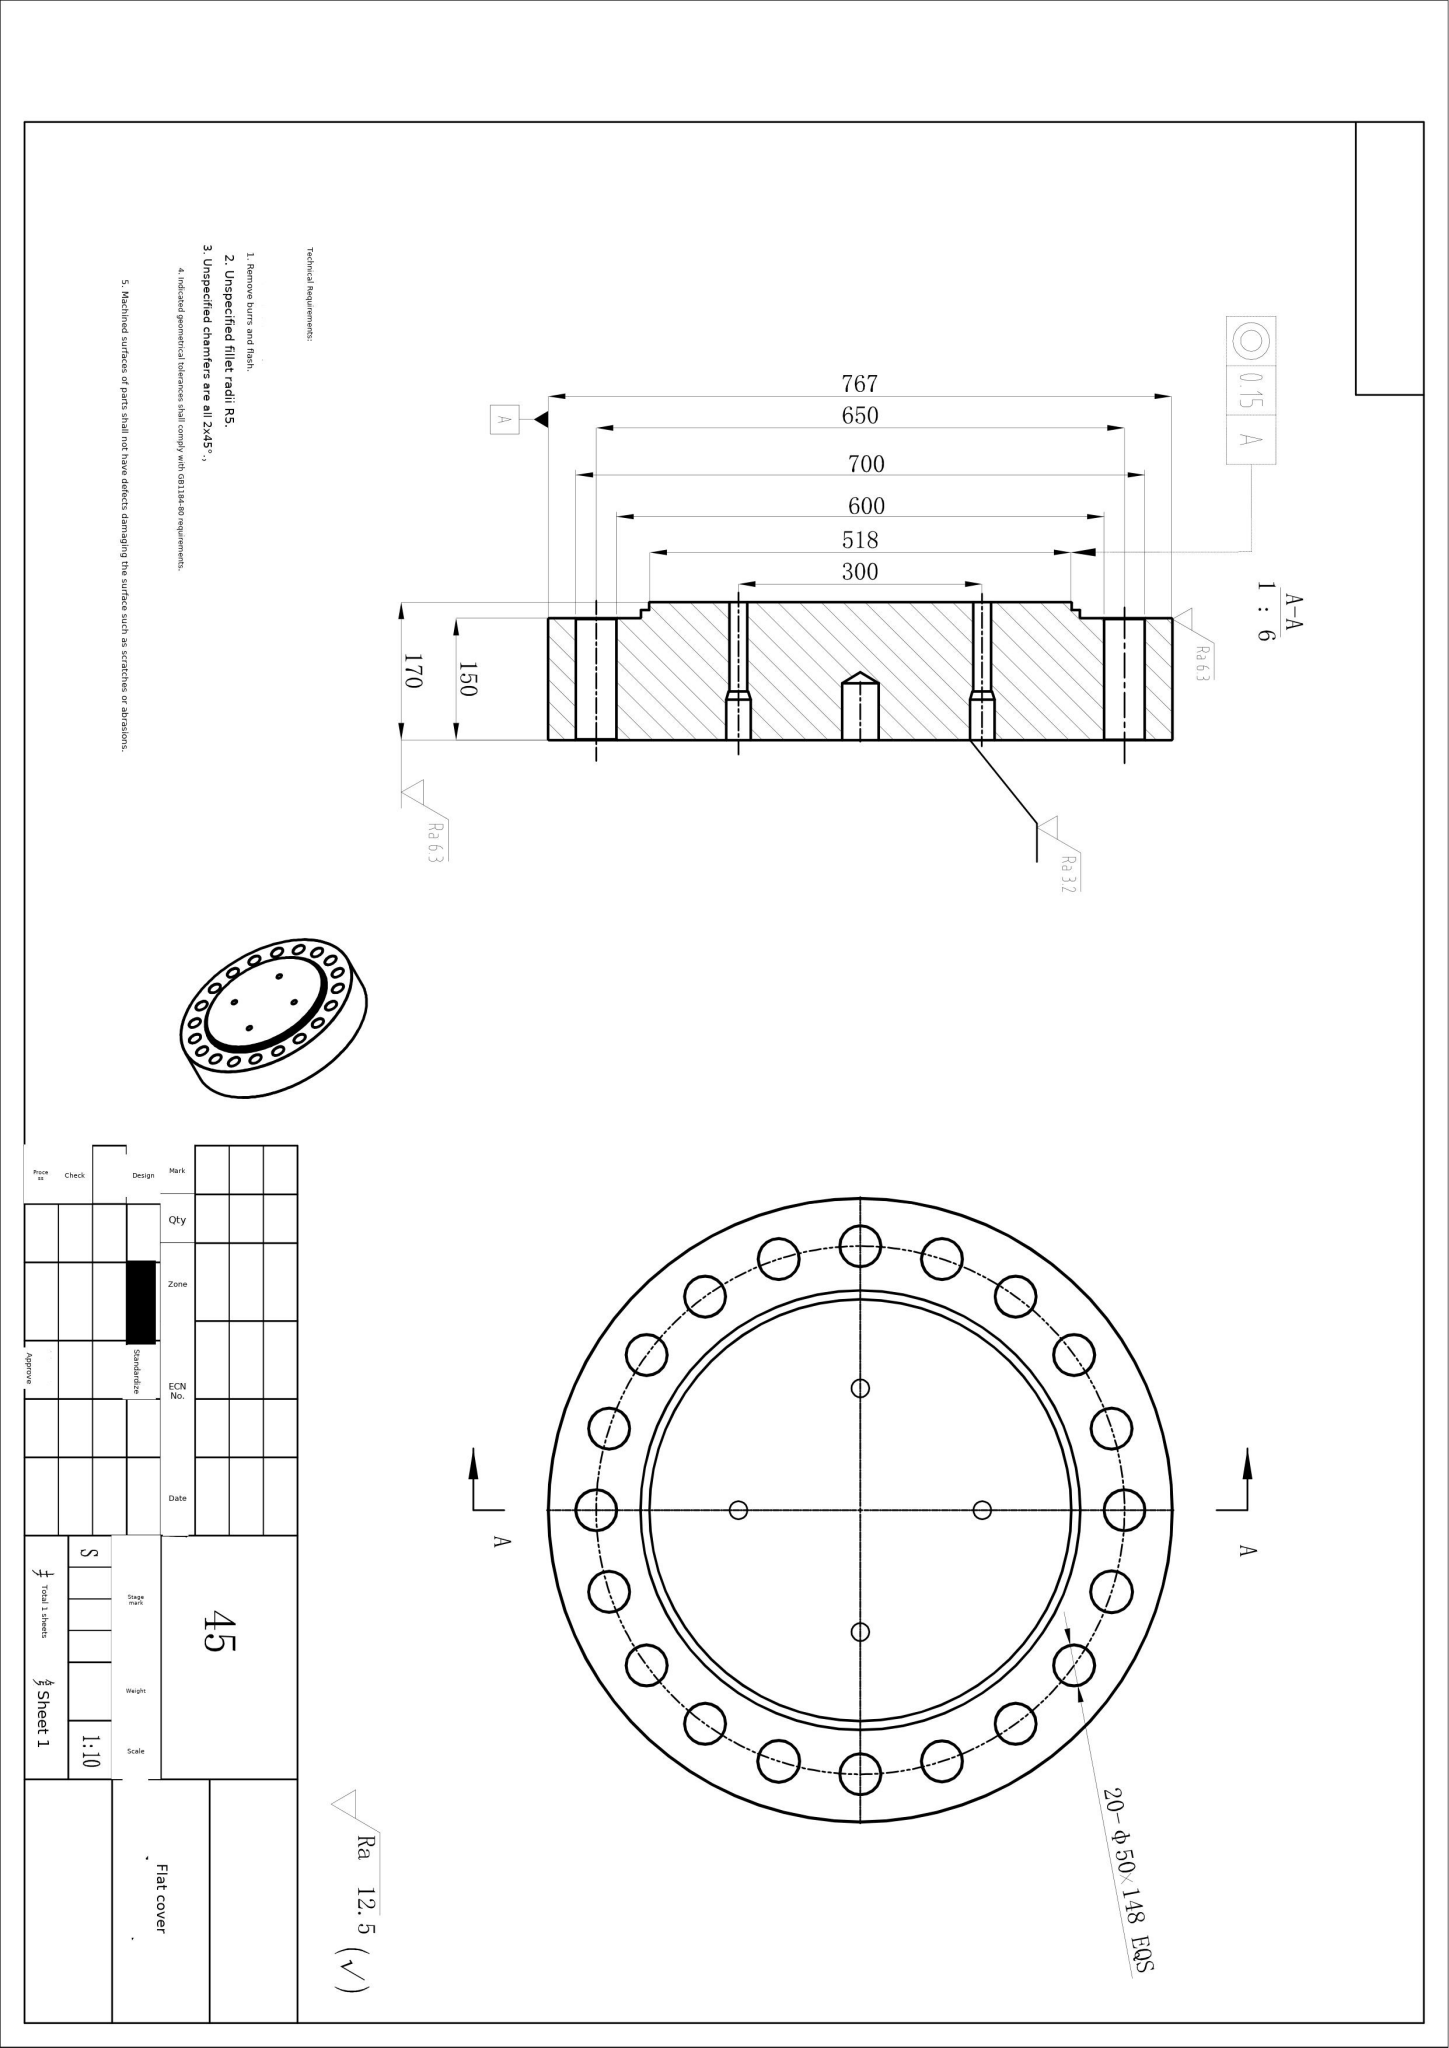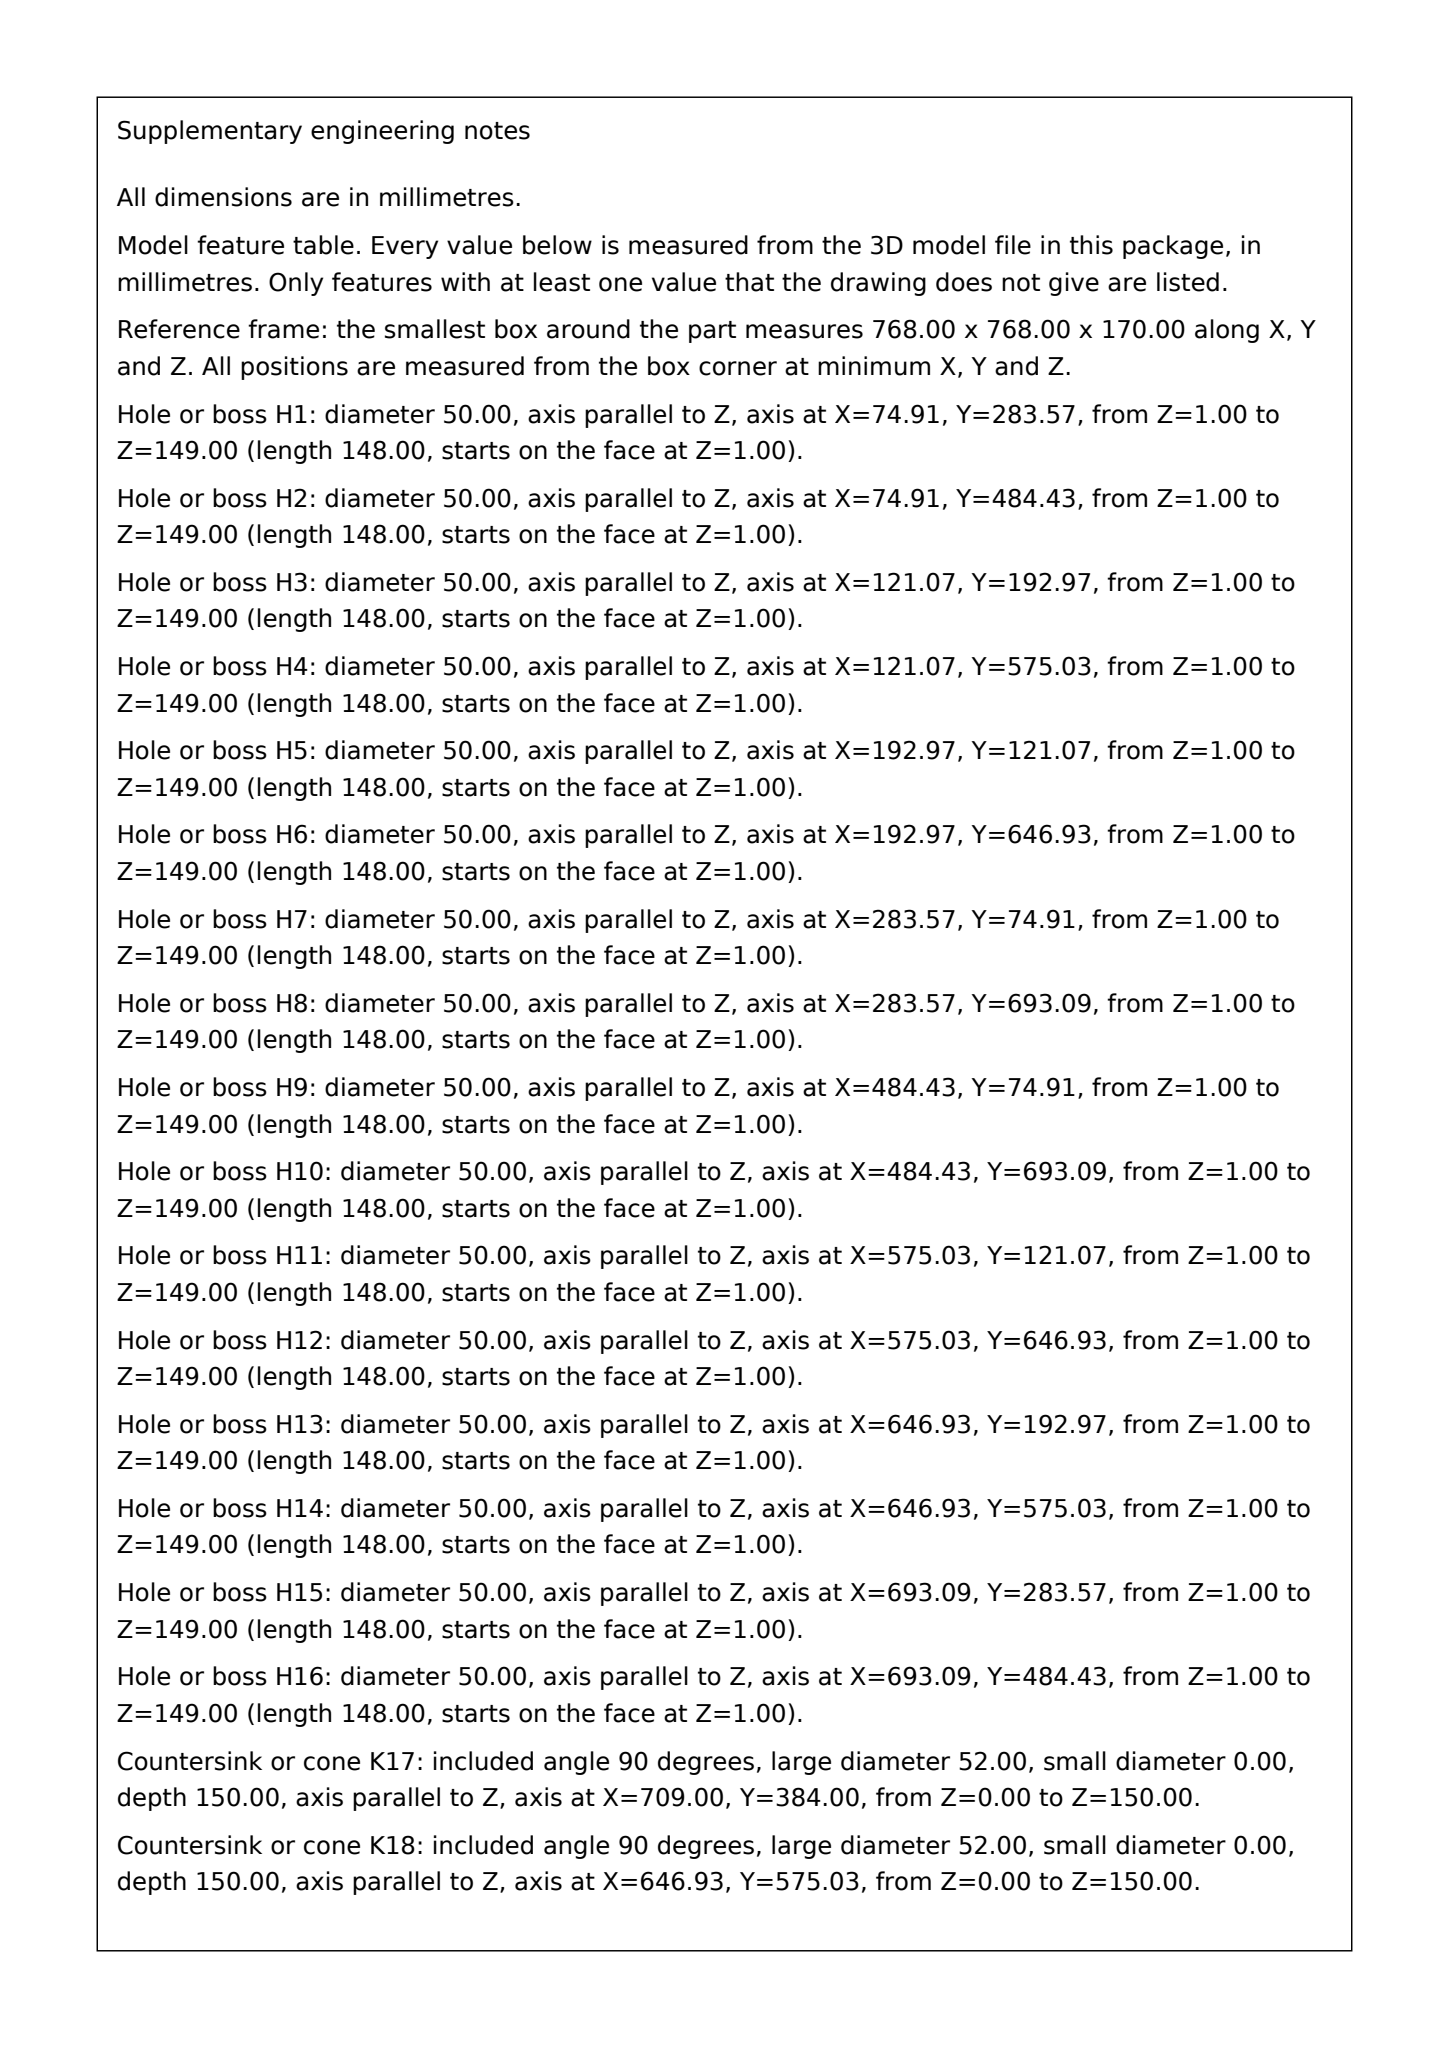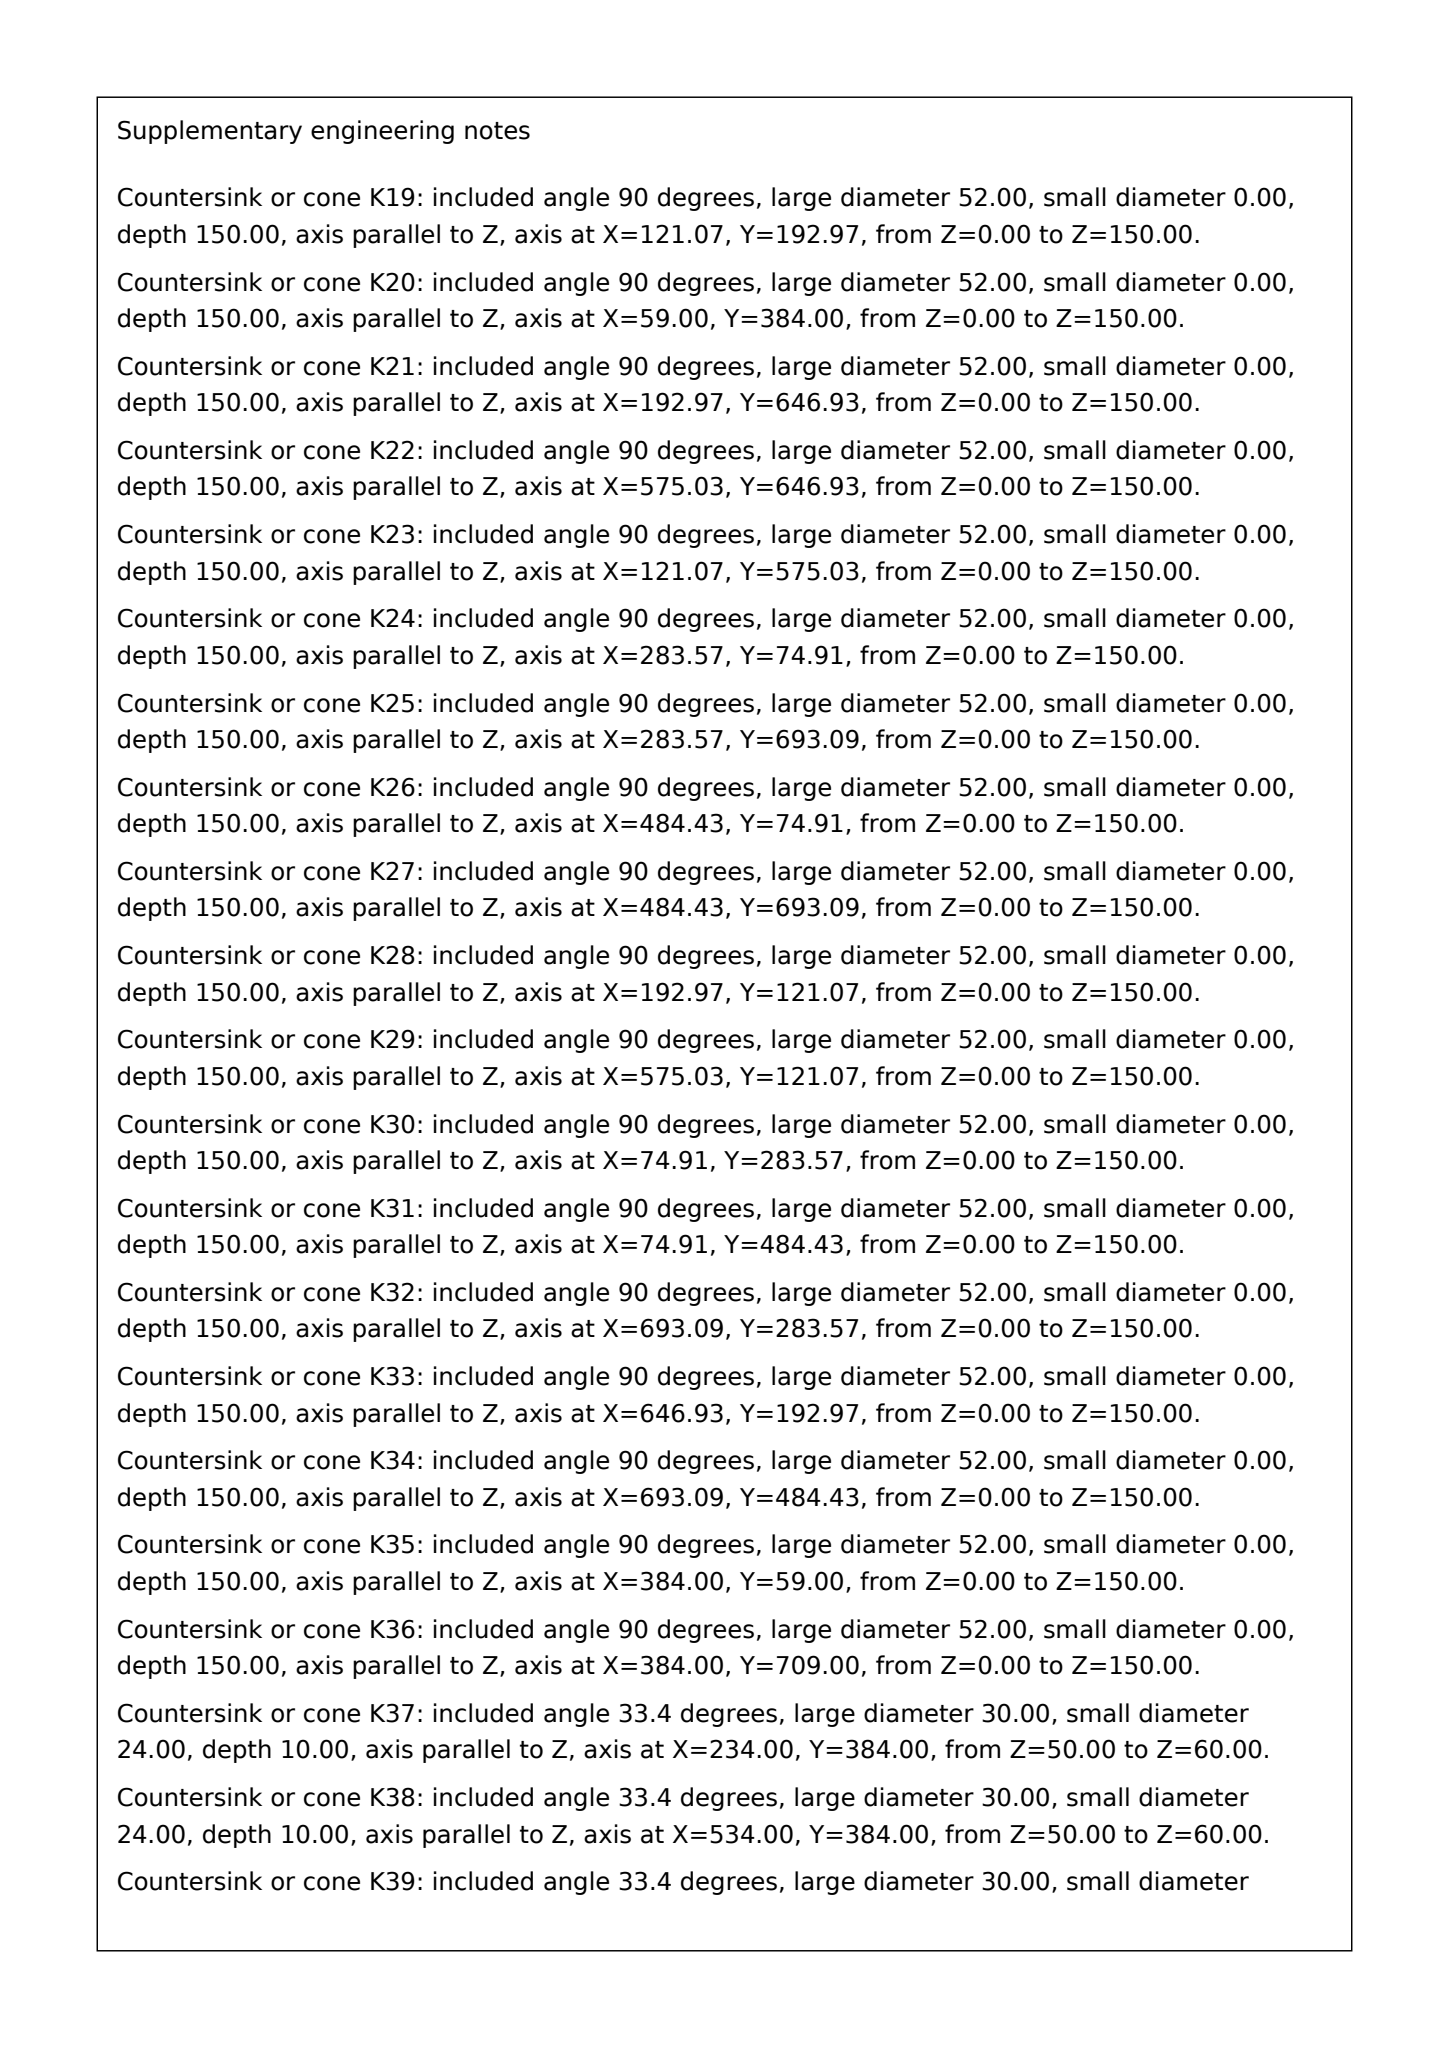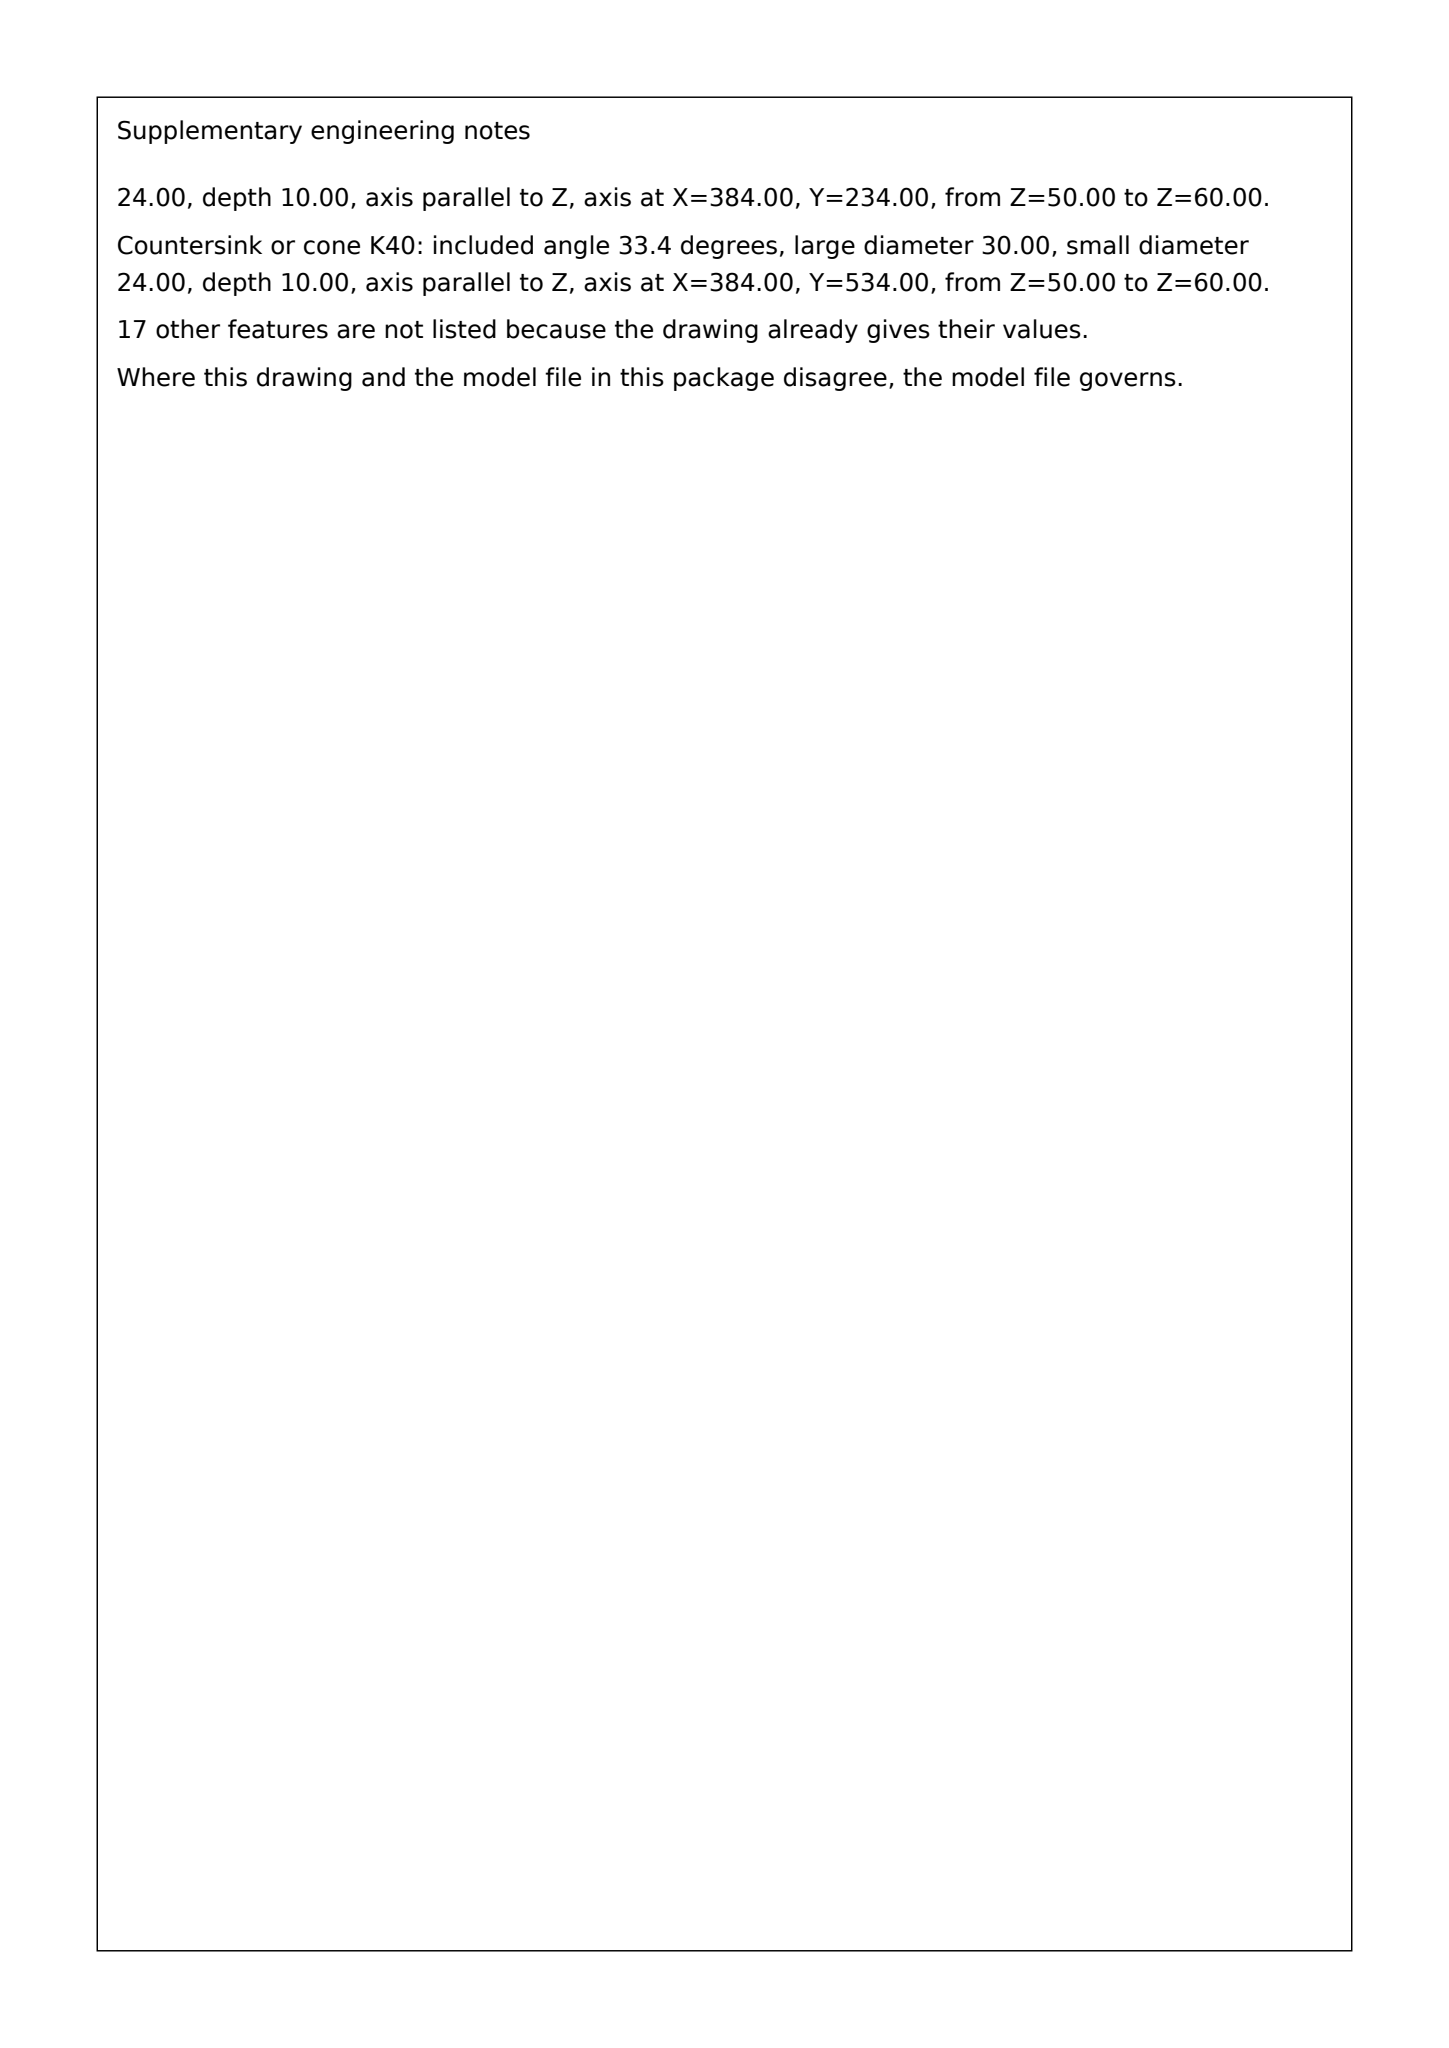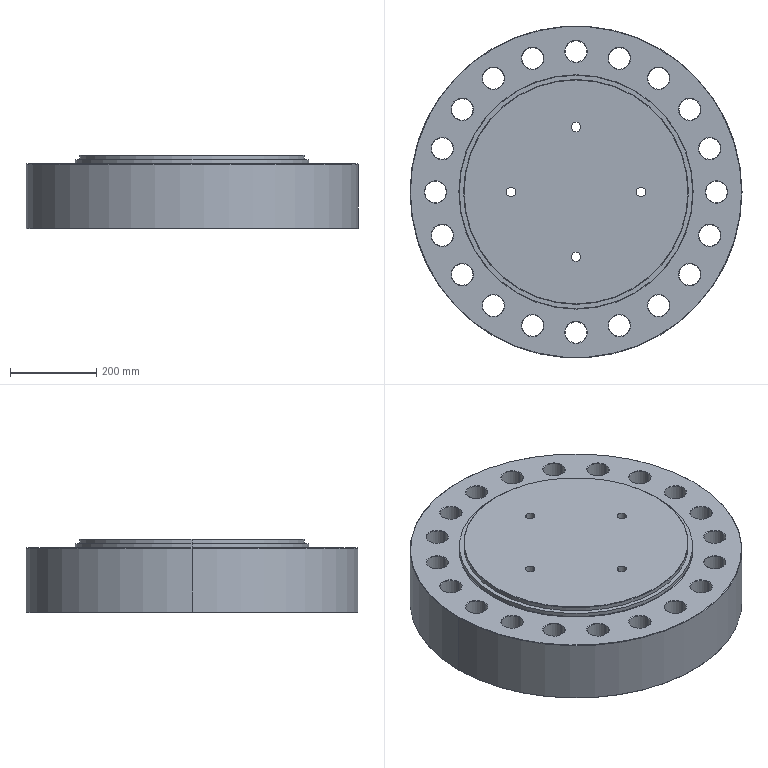Part | SolidWorks | mm | material 45 | 1 solid | 172 faces | box 768 x 768 x 170 mm | volume 67554770 mm3 | cone 100 | cylinder 64 | plane 8 | commonest cylinder face diameters 50 x40 22 x8 30 x8 45 x2 520 x2 540 x2 768 x2
build123d program:
from build123d import *

# Parameters (mm, degrees)
SKETCH1_R                       = 384
BOSS_EXTRUDE1_DEPTH             = 150
SKETCH2_R                       = 270
BOSS_EXTRUDE2_DEPTH             = 10
SKETCH3_R                       = 260
BOSS_EXTRUDE3_DEPTH             = 10
SKETCH4_R                       = 25
CUT_EXTRUDE1_DEPTH              = 432
CHAMFER1_SIZE                   = 1
M42_CLEARANCE_HOLE1_D           = 45
M42_CLEARANCE_HOLE1_DEPTH       = 70
M42_CLEARANCE_HOLE1_CSINK_D     = 45.05
M42_CLEARANCE_HOLE1_CSINK_ANGLE = 90
M42_CLEARANCE_HOLE1_TIP         = 13.519
CIRPATTERN1_COUNT               = 4


with BuildPart() as part:
    # Sketch1 → Boss-Extrude1 (new body)
    with BuildSketch(Plane.XY):
        Circle(SKETCH1_R)
    extrude(amount=BOSS_EXTRUDE1_DEPTH)

    # Sketch2 → Boss-Extrude2 (add)
    with BuildSketch(Plane.XY.offset(150)):
        Circle(SKETCH2_R)
    extrude(amount=BOSS_EXTRUDE2_DEPTH)

    # Sketch3 → Boss-Extrude3 (add)
    with BuildSketch(Plane.XY.offset(160)):
        Circle(SKETCH3_R)
    extrude(amount=BOSS_EXTRUDE3_DEPTH)

    # Sketch4 → Cut-Extrude1 (cut)
    with BuildSketch(Plane(origin=(0, 0, 0), x_dir=(-1, 0, 0), z_dir=(0, 0, -1))):
        with Locations((325, 0)):
            Circle(SKETCH4_R)
        with Locations((309.093, -100.431)):
            Circle(SKETCH4_R)
        with Locations((262.931, -191.03)):
            Circle(SKETCH4_R)
        with Locations((191.03, -262.931)):
            Circle(SKETCH4_R)
        with Locations((100.431, -309.093)):
            Circle(SKETCH4_R)
        with Locations((0, -325)):
            Circle(SKETCH4_R)
        with Locations((-100.431, -309.093)):
            Circle(SKETCH4_R)
        with Locations((-191.03, -262.931)):
            Circle(SKETCH4_R)
        with Locations((-262.931, -191.03)):
            Circle(SKETCH4_R)
        with Locations((-309.093, -100.431)):
            Circle(SKETCH4_R)
        with Locations((-325, 0)):
            Circle(SKETCH4_R)
        with Locations((-309.093, 100.431)):
            Circle(SKETCH4_R)
        with Locations((-262.931, 191.03)):
            Circle(SKETCH4_R)
        with Locations((-191.03, 262.931)):
            Circle(SKETCH4_R)
        with Locations((-100.431, 309.093)):
            Circle(SKETCH4_R)
        with Locations((0, 325)):
            Circle(SKETCH4_R)
        with Locations((100.431, 309.093)):
            Circle(SKETCH4_R)
        with Locations((191.03, 262.931)):
            Circle(SKETCH4_R)
        with Locations((262.931, 191.03)):
            Circle(SKETCH4_R)
        with Locations((309.093, 100.431)):
            Circle(SKETCH4_R)
    extrude(amount=-CUT_EXTRUDE1_DEPTH, mode=Mode.SUBTRACT)

    # Chamfer1
    chamfer1_edges = [part.edges().sort_by_distance(p)[0] for p in [
        (-260, 0, 170),
        (-384, 0, 0),
        (-75.431, 309.093, 150),
        (-75.431, 309.093, 0),
        (25, 325, 150),
        (25, 325, 0),
        (125.431, 309.093, 150),
        (125.431, 309.093, 0),
        (216.03, 262.931, 150),
        (216.03, 262.931, 0),
        (-384, 0, 150),
        (287.931, 191.03, 150),
        (287.931, 191.03, 0),
        (334.093, 100.431, 150),
        (334.093, 100.431, 0),
        (350, 0, 150),
        (350, 0, 0),
        (334.093, -100.431, 150),
        (334.093, -100.431, 0),
        (-270, 0, 150),
        (287.931, -191.03, 150),
        (287.931, -191.03, 0),
        (216.03, -262.931, 150),
        (216.03, -262.931, 0),
        (125.431, -309.093, 150),
        (125.431, -309.093, 0),
        (25, -325, 150),
        (25, -325, 0),
        (-75.431, -309.093, 150),
        (-75.431, -309.093, 0),
        (-166.03, -262.931, 150),
        (-166.03, -262.931, 0),
        (-237.931, -191.03, 150),
        (-237.931, -191.03, 0),
        (-284.093, -100.431, 150),
        (-284.093, -100.431, 0),
        (-166.03, 262.931, 150),
        (-166.03, 262.931, 0),
        (-237.931, 191.03, 150),
        (-237.931, 191.03, 0),
        (-284.093, 100.431, 150),
        (-284.093, 100.431, 0),
        (-300, 0, 150),
        (-300, 0, 0),
    ]]
    chamfer(chamfer1_edges, length=CHAMFER1_SIZE)

    # M42 Clearance Hole1
    with Locations(Plane(origin=(0, 0, 0), x_dir=(-1, 0, 0), z_dir=(0, 0, -1))):
        with Locations((0, 0)):
            CounterSinkHole(M42_CLEARANCE_HOLE1_D / 2, M42_CLEARANCE_HOLE1_CSINK_D / 2, depth=M42_CLEARANCE_HOLE1_DEPTH, counter_sink_angle=M42_CLEARANCE_HOLE1_CSINK_ANGLE)
            with Locations((0, 0, -(M42_CLEARANCE_HOLE1_DEPTH + M42_CLEARANCE_HOLE1_TIP / 2))):  # 118° drill point
                Cone(0, M42_CLEARANCE_HOLE1_D / 2, M42_CLEARANCE_HOLE1_TIP, mode=Mode.SUBTRACT)

    # Sketch14 → Cut-Revolve1 (revolve, cut)
    with BuildSketch(Plane(origin=(0, 0, 0), x_dir=(1, 0, 0), z_dir=(0, 1, 0)), mode=Mode.PRIVATE) as cut_revolve1_sk:
        Polygon((-150, 0), (-135, 0), (-135, -50), (-138, -60), (-139, -60), (-139, -170), (-150, -170), align=None)
    cut_revolve1 = revolve(cut_revolve1_sk.sketch.rotate(Axis((-150, 0, -86.514), (0, 0, 1)), 180), axis=Axis((-150, 0, -86.514), (0, 0, 1)), mode=Mode.SUBTRACT)

    # CirPattern1: Cut-Revolve1 ×4 about axis
    cirpattern1_axis = Axis((0, 0, 0), (0, 0, 1))
    for i in range(1, CIRPATTERN1_COUNT):
        add(cut_revolve1.rotate(cirpattern1_axis, i * 360 / CIRPATTERN1_COUNT), mode=Mode.SUBTRACT)


solid = part.part